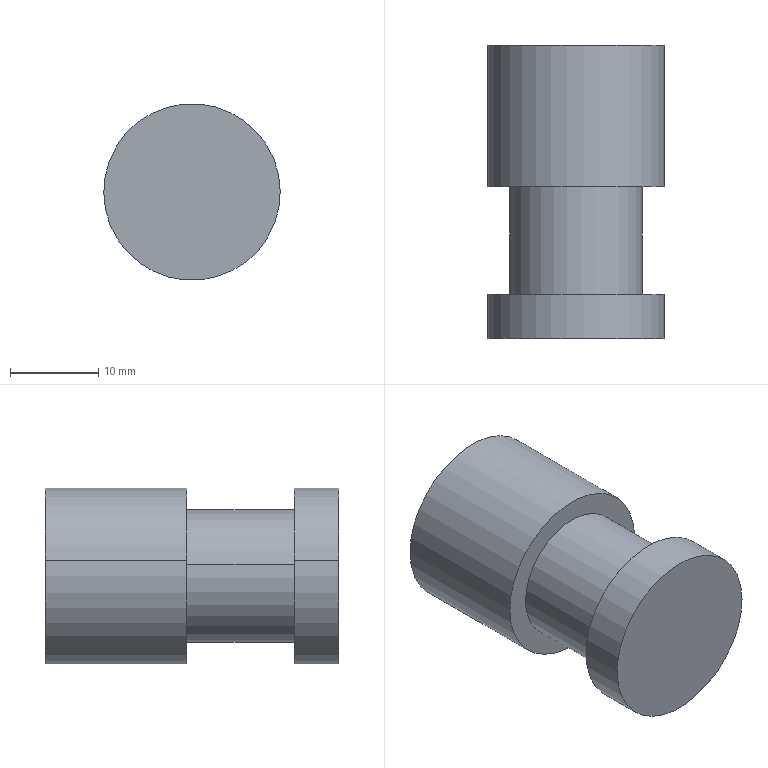Component | SolidWorks | PressingMechanism-31-1 | 1 solid | 14 faces | box 20 x 33.2 x 20 mm | volume 8469 mm3 | cylinder 8 | plane 4 | cone 2 | commonest cylinder face diameters 20 x4 5 x2 15 x2
build123d program:
from build123d import *

# Parameters (mm, degrees)
SKETCH1_R             = 10
EXTRUDE1_DEPTH        = 5
SKETCH2_R             = 7.5
EXTRUDE2_DEPTH        = 12.2
SKETCH3_R             = 10
EXTRUDE3_DEPTH        = 16
M5_TAPPED_HOLE1_D     = 5
M5_TAPPED_HOLE1_DEPTH = 14
M5_TAPPED_HOLE1_TIP   = 1.502


with BuildPart() as part:
    # Sketch1 → Extrude1 (new body)
    with BuildSketch(Plane(origin=(0, 0, 0), x_dir=(0, 0, -1), z_dir=(1, 0, 0))):
        Circle(SKETCH1_R)
    extrude(amount=EXTRUDE1_DEPTH)

    # Sketch2 → Extrude2 (add)
    with BuildSketch(Plane(origin=(5, 0, 0), x_dir=(0, 0, -1), z_dir=(1, 0, 0))):
        Circle(SKETCH2_R)
    extrude(amount=EXTRUDE2_DEPTH)

    # Sketch3 → Extrude3 (add)
    with BuildSketch(Plane(origin=(17.2, 0, 0), x_dir=(0, 0, -1), z_dir=(1, 0, 0))):
        Circle(SKETCH3_R)
    extrude(amount=EXTRUDE3_DEPTH)

    # M5 Tapped Hole1
    with Locations(Plane(origin=(33.2, 0, 0), x_dir=(0, 0, -1), z_dir=(1, 0, 0))):
        with Locations((0, 0)):
            Hole(M5_TAPPED_HOLE1_D / 2, depth=M5_TAPPED_HOLE1_DEPTH)
            with Locations((0, 0, -(M5_TAPPED_HOLE1_DEPTH + M5_TAPPED_HOLE1_TIP / 2))):  # 118° drill point
                Cone(0, M5_TAPPED_HOLE1_D / 2, M5_TAPPED_HOLE1_TIP, mode=Mode.SUBTRACT)


solid = part.part

# Placed as in the assembly
solid = solid.moved(Location((45, -276.2, 55), (0, 0, 90)))
STEP:
#1=CARTESIAN_POINT('',(1.868,-10.118,2.148));
#2=VERTEX_POINT('',#1);
#3=CARTESIAN_POINT('',(1.675,-10.118,2.183));
#4=VERTEX_POINT('',#3);
#5=CARTESIAN_POINT('',(1.772,-10.118,2.165));
#6=DIRECTION('',(0.,1.,0.));
#7=DIRECTION('',(-0.984,0.,0.1784));
#8=AXIS2_PLACEMENT_3D('',#5,#6,#7);
#9=CIRCLE('',#8,0.09843);
#10=EDGE_CURVE('',#2,#4,#9,.T.);
#11=ORIENTED_EDGE('',*,*,#10,.F.);
#12=CARTESIAN_POINT('',(1.868,-9.567,2.148));
#13=VERTEX_POINT('',#12);
#14=CARTESIAN_POINT('',(1.868,-9.567,2.148));
#15=DIRECTION('',(0.,1.,0.));
#16=VECTOR('',#15,39.37);
#17=LINE('',#14,#16);
#18=EDGE_CURVE('',#2,#13,#17,.T.);
#19=ORIENTED_EDGE('',*,*,#18,.T.);
#20=CARTESIAN_POINT('',(1.675,-9.567,2.183));
#21=VERTEX_POINT('',#20);
#22=CARTESIAN_POINT('',(1.772,-9.567,2.165));
#23=DIRECTION('',(0.,1.,0.));
#24=DIRECTION('',(-0.984,0.,0.1784));
#25=AXIS2_PLACEMENT_3D('',#22,#23,#24);
#26=CIRCLE('',#25,0.09843);
#27=EDGE_CURVE('',#13,#21,#26,.T.);
#28=ORIENTED_EDGE('',*,*,#27,.T.);
#29=CARTESIAN_POINT('',(1.675,-9.567,2.183));
#30=DIRECTION('',(0.,1.,0.));
#31=VECTOR('',#30,39.37);
#32=LINE('',#29,#31);
#33=EDGE_CURVE('',#4,#21,#32,.T.);
#34=ORIENTED_EDGE('',*,*,#33,.F.);
#35=EDGE_LOOP('',(#11,#19,#28,#34));
#36=FACE_OUTER_BOUND('',#35,.T.);
#37=CARTESIAN_POINT('',(1.772,-9.567,2.165));
#38=DIRECTION('',(0.,1.,0.));
#39=DIRECTION('',(-0.984,0.,0.1784));
#40=AXIS2_PLACEMENT_3D('',#37,#38,#39);
#41=CYLINDRICAL_SURFACE('',#40,0.09843);
#42=ADVANCED_FACE('',(#36),#41,.F.);
#43=CARTESIAN_POINT('',(1.772,-10.177,2.165));
#44=VERTEX_POINT('',#43);
#45=CARTESIAN_POINT('',(1.675,-10.118,2.183));
#46=DIRECTION('',(-0.8434,0.515,0.1529));
#47=VECTOR('',#46,39.37);
#48=LINE('',#45,#47);
#49=EDGE_CURVE('',#44,#4,#48,.T.);
#50=ORIENTED_EDGE('',*,*,#49,.F.);
#51=CARTESIAN_POINT('',(1.868,-10.118,2.148));
#52=DIRECTION('',(0.8434,0.515,-0.1529));
#53=VECTOR('',#52,39.37);
#54=LINE('',#51,#53);
#55=EDGE_CURVE('',#44,#2,#54,.T.);
#56=ORIENTED_EDGE('',*,*,#55,.T.);
#57=ORIENTED_EDGE('',*,*,#10,.T.);
#58=EDGE_LOOP('',(#50,#56,#57));
#59=FACE_OUTER_BOUND('',#58,.T.);
#60=CARTESIAN_POINT('',(1.772,-10.118,2.165));
#61=DIRECTION('',(0.,1.,0.));
#62=DIRECTION('',(-0.984,0.,0.1784));
#63=AXIS2_PLACEMENT_3D('',#60,#61,#62);
#64=CONICAL_SURFACE('',#63,0.09843,1.03);
#65=ADVANCED_FACE('',(#59),#64,.F.);
#66=CARTESIAN_POINT('',(1.384,-9.567,2.236));
#67=VERTEX_POINT('',#66);
#68=CARTESIAN_POINT('',(2.159,-9.567,2.095));
#69=VERTEX_POINT('',#68);
#70=CARTESIAN_POINT('',(1.772,-9.567,2.165));
#71=DIRECTION('',(0.,1.,0.));
#72=DIRECTION('',(-0.984,0.,0.1784));
#73=AXIS2_PLACEMENT_3D('',#70,#71,#72);
#74=CIRCLE('',#73,0.3937);
#75=EDGE_CURVE('',#67,#69,#74,.T.);
#76=ORIENTED_EDGE('',*,*,#75,.F.);
#77=CARTESIAN_POINT('',(1.384,-10.197,2.236));
#78=VERTEX_POINT('',#77);
#79=CARTESIAN_POINT('',(1.384,-9.567,2.236));
#80=DIRECTION('',(0.,-1.,0.));
#81=VECTOR('',#80,39.37);
#82=LINE('',#79,#81);
#83=EDGE_CURVE('',#67,#78,#82,.T.);
#84=ORIENTED_EDGE('',*,*,#83,.T.);
#85=CARTESIAN_POINT('',(2.159,-10.197,2.095));
#86=VERTEX_POINT('',#85);
#87=CARTESIAN_POINT('',(1.772,-10.197,2.165));
#88=DIRECTION('',(0.,1.,0.));
#89=DIRECTION('',(-0.984,0.,0.1784));
#90=AXIS2_PLACEMENT_3D('',#87,#88,#89);
#91=CIRCLE('',#90,0.3937);
#92=EDGE_CURVE('',#78,#86,#91,.T.);
#93=ORIENTED_EDGE('',*,*,#92,.T.);
#94=CARTESIAN_POINT('',(2.159,-9.567,2.095));
#95=DIRECTION('',(0.,-1.,0.));
#96=VECTOR('',#95,39.37);
#97=LINE('',#94,#96);
#98=EDGE_CURVE('',#69,#86,#97,.T.);
#99=ORIENTED_EDGE('',*,*,#98,.F.);
#100=EDGE_LOOP('',(#76,#84,#93,#99));
#101=FACE_OUTER_BOUND('',#100,.T.);
#102=CARTESIAN_POINT('',(1.772,-9.567,2.165));
#103=DIRECTION('',(0.,-1.,0.));
#104=DIRECTION('',(0.984,0.,-0.1784));
#105=AXIS2_PLACEMENT_3D('',#102,#103,#104);
#106=CYLINDRICAL_SURFACE('',#105,0.3937);
#107=ADVANCED_FACE('',(#101),#106,.T.);
#108=CARTESIAN_POINT('',(1.481,-10.197,2.218));
#109=VERTEX_POINT('',#108);
#110=CARTESIAN_POINT('',(2.062,-10.197,2.113));
#111=VERTEX_POINT('',#110);
#112=CARTESIAN_POINT('',(1.772,-10.197,2.165));
#113=DIRECTION('',(0.,1.,0.));
#114=DIRECTION('',(-0.984,0.,0.1784));
#115=AXIS2_PLACEMENT_3D('',#112,#113,#114);
#116=CIRCLE('',#115,0.2953);
#117=EDGE_CURVE('',#109,#111,#116,.T.);
#118=ORIENTED_EDGE('',*,*,#117,.F.);
#119=CARTESIAN_POINT('',(1.481,-10.677,2.218));
#120=VERTEX_POINT('',#119);
#121=CARTESIAN_POINT('',(1.481,-10.197,2.218));
#122=DIRECTION('',(0.,-1.,0.));
#123=VECTOR('',#122,39.37);
#124=LINE('',#121,#123);
#125=EDGE_CURVE('',#109,#120,#124,.T.);
#126=ORIENTED_EDGE('',*,*,#125,.T.);
#127=CARTESIAN_POINT('',(2.062,-10.677,2.113));
#128=VERTEX_POINT('',#127);
#129=CARTESIAN_POINT('',(1.772,-10.677,2.165));
#130=DIRECTION('',(0.,1.,0.));
#131=DIRECTION('',(-0.984,0.,0.1784));
#132=AXIS2_PLACEMENT_3D('',#129,#130,#131);
#133=CIRCLE('',#132,0.2953);
#134=EDGE_CURVE('',#120,#128,#133,.T.);
#135=ORIENTED_EDGE('',*,*,#134,.T.);
#136=CARTESIAN_POINT('',(2.062,-10.197,2.113));
#137=DIRECTION('',(0.,-1.,0.));
#138=VECTOR('',#137,39.37);
#139=LINE('',#136,#138);
#140=EDGE_CURVE('',#111,#128,#139,.T.);
#141=ORIENTED_EDGE('',*,*,#140,.F.);
#142=EDGE_LOOP('',(#118,#126,#135,#141));
#143=FACE_OUTER_BOUND('',#142,.T.);
#144=CARTESIAN_POINT('',(1.772,-10.197,2.165));
#145=DIRECTION('',(0.,-1.,0.));
#146=DIRECTION('',(0.984,0.,-0.1784));
#147=AXIS2_PLACEMENT_3D('',#144,#145,#146);
#148=CYLINDRICAL_SURFACE('',#147,0.2953);
#149=ADVANCED_FACE('',(#143),#148,.T.);
#150=CARTESIAN_POINT('',(1.384,-10.677,2.236));
#151=VERTEX_POINT('',#150);
#152=CARTESIAN_POINT('',(2.159,-10.677,2.095));
#153=VERTEX_POINT('',#152);
#154=CARTESIAN_POINT('',(1.772,-10.677,2.165));
#155=DIRECTION('',(0.,1.,0.));
#156=DIRECTION('',(-0.984,0.,0.1784));
#157=AXIS2_PLACEMENT_3D('',#154,#155,#156);
#158=CIRCLE('',#157,0.3937);
#159=EDGE_CURVE('',#151,#153,#158,.T.);
#160=ORIENTED_EDGE('',*,*,#159,.F.);
#161=CARTESIAN_POINT('',(1.384,-10.874,2.236));
#162=VERTEX_POINT('',#161);
#163=CARTESIAN_POINT('',(1.384,-10.677,2.236));
#164=DIRECTION('',(0.,-1.,0.));
#165=VECTOR('',#164,39.37);
#166=LINE('',#163,#165);
#167=EDGE_CURVE('',#151,#162,#166,.T.);
#168=ORIENTED_EDGE('',*,*,#167,.T.);
#169=CARTESIAN_POINT('',(2.159,-10.874,2.095));
#170=VERTEX_POINT('',#169);
#171=CARTESIAN_POINT('',(1.772,-10.874,2.165));
#172=DIRECTION('',(0.,1.,0.));
#173=DIRECTION('',(-0.984,0.,0.1784));
#174=AXIS2_PLACEMENT_3D('',#171,#172,#173);
#175=CIRCLE('',#174,0.3937);
#176=EDGE_CURVE('',#162,#170,#175,.T.);
#177=ORIENTED_EDGE('',*,*,#176,.T.);
#178=CARTESIAN_POINT('',(2.159,-10.677,2.095));
#179=DIRECTION('',(0.,-1.,0.));
#180=VECTOR('',#179,39.37);
#181=LINE('',#178,#180);
#182=EDGE_CURVE('',#153,#170,#181,.T.);
#183=ORIENTED_EDGE('',*,*,#182,.F.);
#184=EDGE_LOOP('',(#160,#168,#177,#183));
#185=FACE_OUTER_BOUND('',#184,.T.);
#186=CARTESIAN_POINT('',(1.772,-10.677,2.165));
#187=DIRECTION('',(0.,-1.,0.));
#188=DIRECTION('',(0.984,0.,-0.1784));
#189=AXIS2_PLACEMENT_3D('',#186,#187,#188);
#190=CYLINDRICAL_SURFACE('',#189,0.3937);
#191=ADVANCED_FACE('',(#185),#190,.T.);
#192=CARTESIAN_POINT('',(1.772,-10.677,2.165));
#193=DIRECTION('',(0.,1.,0.));
#194=DIRECTION('',(-0.984,0.,0.1784));
#195=AXIS2_PLACEMENT_3D('',#192,#193,#194);
#196=CIRCLE('',#195,0.3937);
#197=EDGE_CURVE('',#153,#151,#196,.T.);
#198=ORIENTED_EDGE('',*,*,#197,.T.);
#199=ORIENTED_EDGE('',*,*,#159,.T.);
#200=EDGE_LOOP('',(#198,#199));
#201=FACE_OUTER_BOUND('',#200,.T.);
#202=CARTESIAN_POINT('',(1.772,-10.677,2.165));
#203=DIRECTION('',(0.,1.,0.));
#204=DIRECTION('',(-0.984,0.,0.1784));
#205=AXIS2_PLACEMENT_3D('',#202,#203,#204);
#206=CIRCLE('',#205,0.2953);
#207=EDGE_CURVE('',#128,#120,#206,.T.);
#208=ORIENTED_EDGE('',*,*,#207,.F.);
#209=ORIENTED_EDGE('',*,*,#134,.F.);
#210=EDGE_LOOP('',(#208,#209));
#211=FACE_BOUND('',#210,.T.);
#212=CARTESIAN_POINT('',(1.772,-10.677,2.165));
#213=DIRECTION('',(0.,1.,0.));
#214=DIRECTION('',(-0.984,0.,0.1784));
#215=AXIS2_PLACEMENT_3D('',#212,#213,#214);
#216=PLANE('',#215);
#217=ADVANCED_FACE('',(#201,#211),#216,.T.);
#218=ORIENTED_EDGE('',*,*,#167,.F.);
#219=ORIENTED_EDGE('',*,*,#197,.F.);
#220=ORIENTED_EDGE('',*,*,#182,.T.);
#221=CARTESIAN_POINT('',(1.772,-10.874,2.165));
#222=DIRECTION('',(0.,1.,0.));
#223=DIRECTION('',(-0.984,0.,0.1784));
#224=AXIS2_PLACEMENT_3D('',#221,#222,#223);
#225=CIRCLE('',#224,0.3937);
#226=EDGE_CURVE('',#170,#162,#225,.T.);
#227=ORIENTED_EDGE('',*,*,#226,.T.);
#228=EDGE_LOOP('',(#218,#219,#220,#227));
#229=FACE_OUTER_BOUND('',#228,.T.);
#230=CARTESIAN_POINT('',(1.772,-10.677,2.165));
#231=DIRECTION('',(0.,-1.,0.));
#232=DIRECTION('',(0.984,0.,-0.1784));
#233=AXIS2_PLACEMENT_3D('',#230,#231,#232);
#234=CYLINDRICAL_SURFACE('',#233,0.3937);
#235=ADVANCED_FACE('',(#229),#234,.T.);
#236=ORIENTED_EDGE('',*,*,#226,.F.);
#237=ORIENTED_EDGE('',*,*,#176,.F.);
#238=EDGE_LOOP('',(#236,#237));
#239=FACE_OUTER_BOUND('',#238,.T.);
#240=CARTESIAN_POINT('',(1.772,-10.874,2.165));
#241=DIRECTION('',(0.,1.,0.));
#242=DIRECTION('',(-0.984,0.,0.1784));
#243=AXIS2_PLACEMENT_3D('',#240,#241,#242);
#244=PLANE('',#243);
#245=ADVANCED_FACE('',(#239),#244,.F.);
#246=ORIENTED_EDGE('',*,*,#125,.F.);
#247=CARTESIAN_POINT('',(1.772,-10.197,2.165));
#248=DIRECTION('',(0.,1.,0.));
#249=DIRECTION('',(-0.984,0.,0.1784));
#250=AXIS2_PLACEMENT_3D('',#247,#248,#249);
#251=CIRCLE('',#250,0.2953);
#252=EDGE_CURVE('',#111,#109,#251,.T.);
#253=ORIENTED_EDGE('',*,*,#252,.F.);
#254=ORIENTED_EDGE('',*,*,#140,.T.);
#255=ORIENTED_EDGE('',*,*,#207,.T.);
#256=EDGE_LOOP('',(#246,#253,#254,#255));
#257=FACE_OUTER_BOUND('',#256,.T.);
#258=CARTESIAN_POINT('',(1.772,-10.197,2.165));
#259=DIRECTION('',(0.,-1.,0.));
#260=DIRECTION('',(0.984,0.,-0.1784));
#261=AXIS2_PLACEMENT_3D('',#258,#259,#260);
#262=CYLINDRICAL_SURFACE('',#261,0.2953);
#263=ADVANCED_FACE('',(#257),#262,.T.);
#264=CARTESIAN_POINT('',(1.772,-10.197,2.165));
#265=DIRECTION('',(0.,1.,0.));
#266=DIRECTION('',(-0.984,0.,0.1784));
#267=AXIS2_PLACEMENT_3D('',#264,#265,#266);
#268=CIRCLE('',#267,0.3937);
#269=EDGE_CURVE('',#86,#78,#268,.T.);
#270=ORIENTED_EDGE('',*,*,#269,.F.);
#271=ORIENTED_EDGE('',*,*,#92,.F.);
#272=EDGE_LOOP('',(#270,#271));
#273=FACE_OUTER_BOUND('',#272,.T.);
#274=ORIENTED_EDGE('',*,*,#252,.T.);
#275=ORIENTED_EDGE('',*,*,#117,.T.);
#276=EDGE_LOOP('',(#274,#275));
#277=FACE_BOUND('',#276,.T.);
#278=CARTESIAN_POINT('',(1.772,-10.197,2.165));
#279=DIRECTION('',(0.,1.,0.));
#280=DIRECTION('',(-0.984,0.,0.1784));
#281=AXIS2_PLACEMENT_3D('',#278,#279,#280);
#282=PLANE('',#281);
#283=ADVANCED_FACE('',(#273,#277),#282,.F.);
#284=ORIENTED_EDGE('',*,*,#83,.F.);
#285=CARTESIAN_POINT('',(1.772,-9.567,2.165));
#286=DIRECTION('',(0.,1.,0.));
#287=DIRECTION('',(-0.984,0.,0.1784));
#288=AXIS2_PLACEMENT_3D('',#285,#286,#287);
#289=CIRCLE('',#288,0.3937);
#290=EDGE_CURVE('',#69,#67,#289,.T.);
#291=ORIENTED_EDGE('',*,*,#290,.F.);
#292=ORIENTED_EDGE('',*,*,#98,.T.);
#293=ORIENTED_EDGE('',*,*,#269,.T.);
#294=EDGE_LOOP('',(#284,#291,#292,#293));
#295=FACE_OUTER_BOUND('',#294,.T.);
#296=CARTESIAN_POINT('',(1.772,-9.567,2.165));
#297=DIRECTION('',(0.,-1.,0.));
#298=DIRECTION('',(0.984,0.,-0.1784));
#299=AXIS2_PLACEMENT_3D('',#296,#297,#298);
#300=CYLINDRICAL_SURFACE('',#299,0.3937);
#301=ADVANCED_FACE('',(#295),#300,.T.);
#302=CARTESIAN_POINT('',(1.772,-9.567,2.165));
#303=DIRECTION('',(0.,1.,0.));
#304=DIRECTION('',(-0.984,0.,0.1784));
#305=AXIS2_PLACEMENT_3D('',#302,#303,#304);
#306=CIRCLE('',#305,0.09843);
#307=EDGE_CURVE('',#21,#13,#306,.T.);
#308=ORIENTED_EDGE('',*,*,#307,.F.);
#309=ORIENTED_EDGE('',*,*,#27,.F.);
#310=EDGE_LOOP('',(#308,#309));
#311=FACE_BOUND('',#310,.T.);
#312=ORIENTED_EDGE('',*,*,#290,.T.);
#313=ORIENTED_EDGE('',*,*,#75,.T.);
#314=EDGE_LOOP('',(#312,#313));
#315=FACE_OUTER_BOUND('',#314,.T.);
#316=CARTESIAN_POINT('',(1.772,-9.567,2.165));
#317=DIRECTION('',(0.,1.,0.));
#318=DIRECTION('',(-0.984,0.,0.1784));
#319=AXIS2_PLACEMENT_3D('',#316,#317,#318);
#320=PLANE('',#319);
#321=ADVANCED_FACE('',(#311,#315),#320,.T.);
#322=ORIENTED_EDGE('',*,*,#55,.F.);
#323=ORIENTED_EDGE('',*,*,#49,.T.);
#324=CARTESIAN_POINT('',(1.772,-10.118,2.165));
#325=DIRECTION('',(0.,1.,0.));
#326=DIRECTION('',(-0.984,0.,0.1784));
#327=AXIS2_PLACEMENT_3D('',#324,#325,#326);
#328=CIRCLE('',#327,0.09843);
#329=EDGE_CURVE('',#4,#2,#328,.T.);
#330=ORIENTED_EDGE('',*,*,#329,.T.);
#331=EDGE_LOOP('',(#322,#323,#330));
#332=FACE_OUTER_BOUND('',#331,.T.);
#333=CARTESIAN_POINT('',(1.772,-10.118,2.165));
#334=DIRECTION('',(0.,1.,0.));
#335=DIRECTION('',(-0.984,0.,0.1784));
#336=AXIS2_PLACEMENT_3D('',#333,#334,#335);
#337=CONICAL_SURFACE('',#336,0.09843,1.03);
#338=ADVANCED_FACE('',(#332),#337,.F.);
#339=ORIENTED_EDGE('',*,*,#18,.F.);
#340=ORIENTED_EDGE('',*,*,#329,.F.);
#341=ORIENTED_EDGE('',*,*,#33,.T.);
#342=ORIENTED_EDGE('',*,*,#307,.T.);
#343=EDGE_LOOP('',(#339,#340,#341,#342));
#344=FACE_OUTER_BOUND('',#343,.T.);
#345=CARTESIAN_POINT('',(1.772,-9.567,2.165));
#346=DIRECTION('',(0.,1.,0.));
#347=DIRECTION('',(-0.984,0.,0.1784));
#348=AXIS2_PLACEMENT_3D('',#345,#346,#347);
#349=CYLINDRICAL_SURFACE('',#348,0.09843);
#350=ADVANCED_FACE('',(#344),#349,.F.);
#351=CLOSED_SHELL('',(#42,#65,#107,#149,#191,#217,#235,#245,#263,#283,#301,#321,#338,#350));
#352=MANIFOLD_SOLID_BREP('',#351);
#353=CARTESIAN_POINT('',(0.,0.,0.));
#354=DIRECTION('',(0.,0.,1.));
#355=DIRECTION('',(1.,0.,0.));
#356=AXIS2_PLACEMENT_3D('',#353,#354,#355);
#357=(LENGTH_UNIT()NAMED_UNIT(*)SI_UNIT($,.METRE.));
#358=LENGTH_MEASURE_WITH_UNIT(LENGTH_MEASURE(0.0254),#357);
#359=DIMENSIONAL_EXPONENTS(1.,0.,0.,0.,0.,0.,0.);
#360=(CONVERSION_BASED_UNIT('',#358)LENGTH_UNIT()NAMED_UNIT(#359));
#361=UNCERTAINTY_MEASURE_WITH_UNIT(LENGTH_MEASURE(0.00001),#360,'','');
#362=(NAMED_UNIT(*)PLANE_ANGLE_UNIT()SI_UNIT($,.RADIAN.));
#363=(NAMED_UNIT(*)SI_UNIT($,.STERADIAN.)SOLID_ANGLE_UNIT());
#364=(GEOMETRIC_REPRESENTATION_CONTEXT(3)GLOBAL_UNCERTAINTY_ASSIGNED_CONTEXT((#361))GLOBAL_UNIT_ASSIGNED_CONTEXT((#360,#362,#363))REPRESENTATION_CONTEXT('',''));
#365=ADVANCED_BREP_SHAPE_REPRESENTATION('',(#352,#356),#364);
#366=COLOUR_RGB('',0.7922,0.8196,0.9333);
#367=FILL_AREA_STYLE_COLOUR('',#366);
#368=FILL_AREA_STYLE('',(#367));
#369=SURFACE_STYLE_FILL_AREA(#368);
#370=SURFACE_SIDE_STYLE('',(#369));
#371=SURFACE_STYLE_USAGE(.BOTH.,#370);
#372=PRESENTATION_STYLE_ASSIGNMENT((#371));
#373=STYLED_ITEM('',(#372),#352);
#374=PRESENTATION_LAYER_ASSIGNMENT('','',(#373));
#375=(LENGTH_UNIT()NAMED_UNIT(*)SI_UNIT($,.METRE.));
#376=LENGTH_MEASURE_WITH_UNIT(LENGTH_MEASURE(0.0254),#375);
#377=DIMENSIONAL_EXPONENTS(1.,0.,0.,0.,0.,0.,0.);
#378=(CONVERSION_BASED_UNIT('',#376)LENGTH_UNIT()NAMED_UNIT(#377));
#379=UNCERTAINTY_MEASURE_WITH_UNIT(LENGTH_MEASURE(0.00001),#378,'','');
#380=(NAMED_UNIT(*)PLANE_ANGLE_UNIT()SI_UNIT($,.RADIAN.));
#381=(NAMED_UNIT(*)SI_UNIT($,.STERADIAN.)SOLID_ANGLE_UNIT());
#382=(GEOMETRIC_REPRESENTATION_CONTEXT(3)GLOBAL_UNCERTAINTY_ASSIGNED_CONTEXT((#379))GLOBAL_UNIT_ASSIGNED_CONTEXT((#378,#380,#381))REPRESENTATION_CONTEXT('',''));
#383=MECHANICAL_DESIGN_GEOMETRIC_PRESENTATION_REPRESENTATION('',(#373),#382);